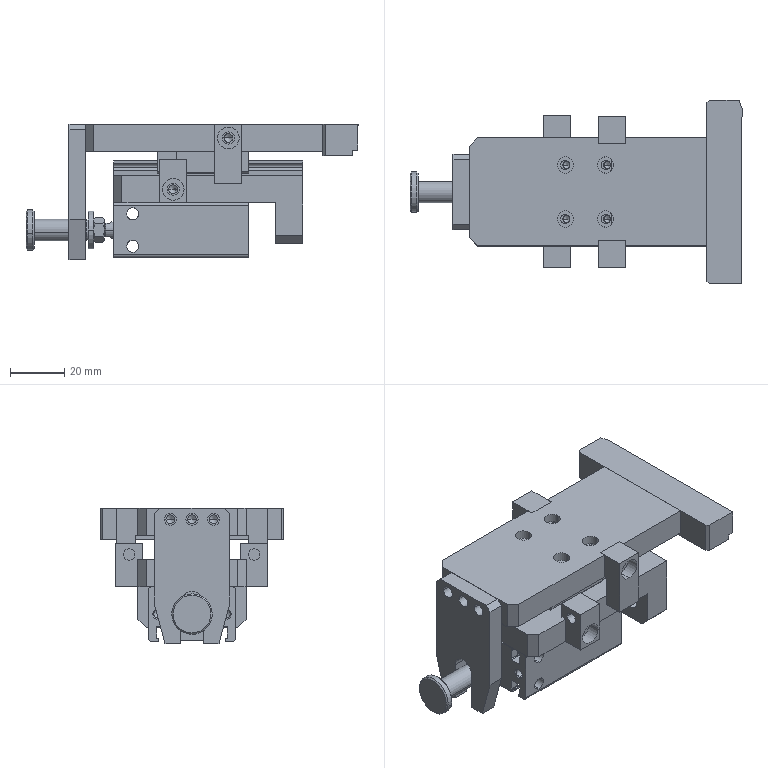Assembly | SolidWorks | mm | 15 component files | 15 solids | 718 faces | box 122.92 x 68 x 50 mm | volume 118126 mm3 | plane 338 | cylinder 281 | cone 99 | commonest cylinder face diameters 0.4 x40 4.5 x34 3.3 x22 2.5 x18 6 x18 8 x16 0.8 x16 2 x12
Bill of materials:
09b_SEB13 | 1 |  | Rectangular block with an inverted-U (channel) cross-section, a central body and a separate end section at each end, four counterbored holes on the top, and holes in the end face; looks like a linear-guide carriage block.
09HHHHH1 | 1 |  | Long rectangular bar with two round through holes in one long side face, a chamfer on one end, and a small step at one corner.
09HHHHH3 | 1 |  | Rectangular plate with four counterbored holes in a rectangular pattern, rectangular side notches at mid-length, chamfered corners at one end, and a wide shallow rebate along the underside.
09HHHHHH2 | 1 |  | Stepped rectangular block with an L-shaped side profile, a narrow slot running along the top, side notches, several small holes on top, and three larger holes in one end face.
09HHHHHH4 | 1 |  | Flat fork-shaped plate with three round holes in a row near the top edge, chamfered top corners, and a U-shaped slot open at the bottom between two tapered legs.
09HHHHHH5 | 1 |  | Flanged cylindrical sleeve/pin: a round flange with chamfered edges and a longer cylindrical shank with a chamfered end, plus an axial bore.
09HHHHHH6 | 1 |  | Flat annular ring (plain washer shape) with a concentric round hole and uniform thickness.
09HHHHHH7 | 2 |  | Long straight bar with a roughly rectangular cross-section, a semicircular groove along each side face, and three counterbored holes spaced along the top; looks like a linear guide rail.
09HHHHHH8 | 2 |  | Small rectangular block with an L-shaped (stepped) profile and one round through hole crossing the upper, wider section.
09r_SEB13_70 | 1 |  | Rectangular block with two round through holes at right angles to each other, set at different heights on adjacent side faces.
Mates:
1. coincident | 09HHHHH1-1 face at (-0.5807, 7.617, 8.844) dir (0, 0, 1) | 09HHHHH3-1 face at (-650.94, -266.383, 8.844) dir (0, 0, 1)
2. coincident | 09HHHHH1-1 face at (-562.94, -320.383, 8.844) dir (-1, 0, 0) | 09HHHHH3-1 face at (-562.94, 14.788, 6.765) dir (1, 0, 0)
3. coincident | 09HHHHHH2-1 face at (-570.359, -280.383, -12.156) dir (0, 0, 1) | 09r_SEB13_70-1 face at (-640.359, -280.883, -12.156) dir (0, 0, -1)
4. coincident | 09HHHHHH2-1 face at (-570.359, -292.383, -10.156) dir (0, 1, 0) | 09r_SEB13_70-1 face at (-640.359, -292.383, -11.656) dir (0, -1, 0)
5. coincident | 09HHHHHH2-1 face at (-640.359, -306.383, -20.156) dir (0, 0, -1) | 09MD-16x10-S (0)-1/09MD 16x10-S10 - Body-1 face at (-590.359, -299.033, -20.156) dir (0, 0, 1)
6. coincident | 09HHHHHH2-1 face at (-640.359, -306.383, -10.156) dir (-1, 0, 0) | 09MD-16x10-S (0)-1/09MD 16x10-S10 - Body-1 face at (-640.359, -299.033, -20.356) dir (-1, 0, 0)
7. distance | 09MD-16x10-S (0)-1/09MD 16x10-S10 - Body-1 face at (-590.359, -270.283, -39.356) dir (0, 1, 0) | 09HHHHHH2-1 face at (-8, -266.383, 6.344) dir (0, 1, 0)
8. concentric | 09HHHHHH2-1 face at (-618.359, -306.383, -15.156) dir (0, -1, 0) r 1.65 | 09HHHHHH8-2 face at (-618.359, -314.383, -15.156) dir (0, -1, 0) r 2.25
9. coincident | 09HHHHHH2-1 face at (-613.359, -304.383, -35.156) dir (0, -1, 0) | 09HHHHHH8-2 face at (-1228.718, -304.383, 6.344) dir (0, 1, 0)
10. coincident | 09HHHHHH2-1 face at (-623.359, -306.383, -35.156) dir (1, 0, 0) | 09HHHHHH8-2 face at (-623.359, -314.383, -10.156) dir (-1, 0, 0)
11. coincident | 09HHHHH3-1 face at (-562.94, -272.883, 0.8438) dir (0, 0, -1) | 09b_SEB13-1 face at (-617.259, -280.133, 0.8438) dir (0, 0, 1)
12. coincident | 09HHHHH3-1 face at (-562.94, -272.883, -1.156) dir (0, -1, 0) | 09b_SEB13-1 face at (-617.259, -272.883, 0.3438) dir (0, 1, 0)
13. distance | 09HHHHHH4-1 face at (-656.94, -272.383, 8.844) dir (0, 1, 0) | 09HHHHH3-1 face at (-650.94, -266.383, 8.844) dir (0, 1, 0)
14. coincident | 09HHHHH3-1 face at (-650.94, 14.788, 6.765) dir (-1, 0, 0) | 09HHHHHH4-1 face at (-650.94, 19.683, 6.344) dir (1, 0, 0)
15. coincident | 09HHHHH3-1 face at (-650.94, -266.383, 8.844) dir (0, 0, 1) | 09HHHHHH4-1 face at (-656.94, -272.383, 8.844) dir (0, 0, 1)
16. coincident | 09HHHHH3-1 face at (-650.94, -266.383, 8.844) dir (0, 0, 1) | 09HHHHHH7-1 face at (-10.581, 13.617, 8.844) dir (0, 0, 1)
17. coincident | 09HHHHH3-1 face at (-592.94, -268.383, -1.156) dir (0, 1, 0) | 09HHHHHH7-1 face at (-592.94, -268.383, -21.156) dir (0, -1, 0)
18. coincident | 09HHHHH3-1 face at (-592.94, -266.383, -1.156) dir (-1, 0, 0) | 09HHHHHH7-1 face at (-592.94, -268.383, -21.156) dir (1, 0, 0)
19. coincident | 09HHHHH3-1 face at (-592.94, -304.383, -1.156) dir (0, -1, 0) | 09HHHHHH7-2 face at (-602.94, -304.383, -21.156) dir (0, 1, 0)
20. coincident | 09HHHHH3-1 face at (-592.94, -306.383, -1.156) dir (-1, 0, 0) | 09HHHHHH7-2 face at (-592.94, -304.383, -21.156) dir (1, 0, 0)
21. coincident | 09HHHHH3-1 face at (-650.94, -266.383, 8.844) dir (0, 0, 1) | 09HHHHHH7-2 face at (-1185.298, -586.383, 8.844) dir (0, 0, 1)
22. coincident | 09r_SEB13_70-1 axis at (-651.259, -286.383, -4.656) dir (1, 0, 0) | 09b_SEB13-1 axis at (-688.209, -286.383, -4.656) dir (1, 0, 0)
23. coincident | 09r_SEB13_70-1 axis at (-651.259, -286.383, -4.656) dir (1, 0, 0) | 09b_SEB13-1 axis at (-688.209, -286.383, -4.656) dir (1, 0, 0)
24. coincident | 09r_SEB13_70-1 axis at (-651.259, -286.383, -4.656) dir (1, 0, 0) | 09b_SEB13-1 axis at (-688.209, -286.383, -4.656) dir (1, 0, 0)
25. angle | 09b_SEB13-1 plane at (-607.309, -286.383, -9.156) dir (0, -1, 0) | 09r_SEB13_70-1 plane at (-570.359, -286.383, -12.156) dir (0, -1, 0)
26. concentric | 09MD-16x10-S (0)-1/09MD 16x10-S10 - Rod-1 face at (-599.359, -286.383, -30.256) dir (-1, 0, 0) r 2.5 | 09HHHHHH5-1 face at (-669.859, -286.383, -30.256) dir (1, 0, 0) r 4
27. concentric | 09MD-16x10-S (0)-1/09MD 16x10-S10 - Rod-1 face at (-599.359, -286.383, -30.256) dir (-1, 0, 0) r 2.5 | 09HHHHHH6-1 face at (-649.859, -286.383, -30.256) dir (1, 0, 0) r 2.75
28. coincident | 09MD-16x10-S (0)-1/09MD 16x10 - Nut Rod-1 face at (-647.859, -286.383, -34.256) dir (-1, 0, 0) | 09HHHHHH6-1 face at (-647.859, -286.383, -30.256) dir (1, 0, 0)
29. coincident | 09HHHHHH5-1 face at (-649.859, -286.383, -30.256) dir (1, 0, 0) | 09HHHHHH6-1 face at (-649.859, -286.383, -30.256) dir (-1, 0, 0)
30. width | 09HHHHH3-1 face at (-650.94, -306.383, 8.844) dir (0, -1, 0) | 09HHHHH3-1 face at (-650.94, -266.383, 8.844) dir (0, 1, 0) | 09HHHHH1-1 face at (-562.94, -252.383, 8.844) dir (0, 1, 0) | 09HHHHH1-1 face at (-562.94, -320.383, 8.844) dir (0, -1, 0)
31. concentric | 09HHHHHH2-1 face at (-618.359, -268.383, -15.156) dir (0, 1, 0) r 1.65 | 09HHHHHH8-1 face at (-618.359, -258.084, -15.156) dir (0, 1, 0) r 2.25
32. coincident | 09MD 16x10-S10 - Body-1 axis at (80.9, 0, 0) dir (-1, 0, 0) | 09MD 16x10-S10 - Rod-1 axis at (80.9, 0, 0) dir (-1, 0, 0)
33. angle | 09MD 16x10-S10 - Rod-1 plane at (0, 0, 0) dir (0, 1, 0) | 09MD 16x10-S10 - Body-1 plane at (0, 0, 0) dir (0, 0, -1)
34. coincident | 09MD 16x10-S10 - Rod-1 axis at (-80.9, 0, 0) dir (1, 0, 0) | 09MD 16x10 - Nut Rod-1 axis at (-84.4, 0, 0) dir (1, 0, 0)
35. angle | 09MD 16x10 - Nut Rod-1 plane at (-3.5, 0, 0) dir (0, 1, 0) | 09MD 16x10-S10 - Rod-1 plane at (0, 0, 0) dir (0, 1, 0)
36. coincident | 09MD 16x10-S10 - Rod-1 edge at (-3.5, 0, 0) dir (-1, 0, 0) r 2.4 | 09MD 16x10 - Nut Rod-1 face at (-3.5, 0, 0) dir (1, 0, 0)